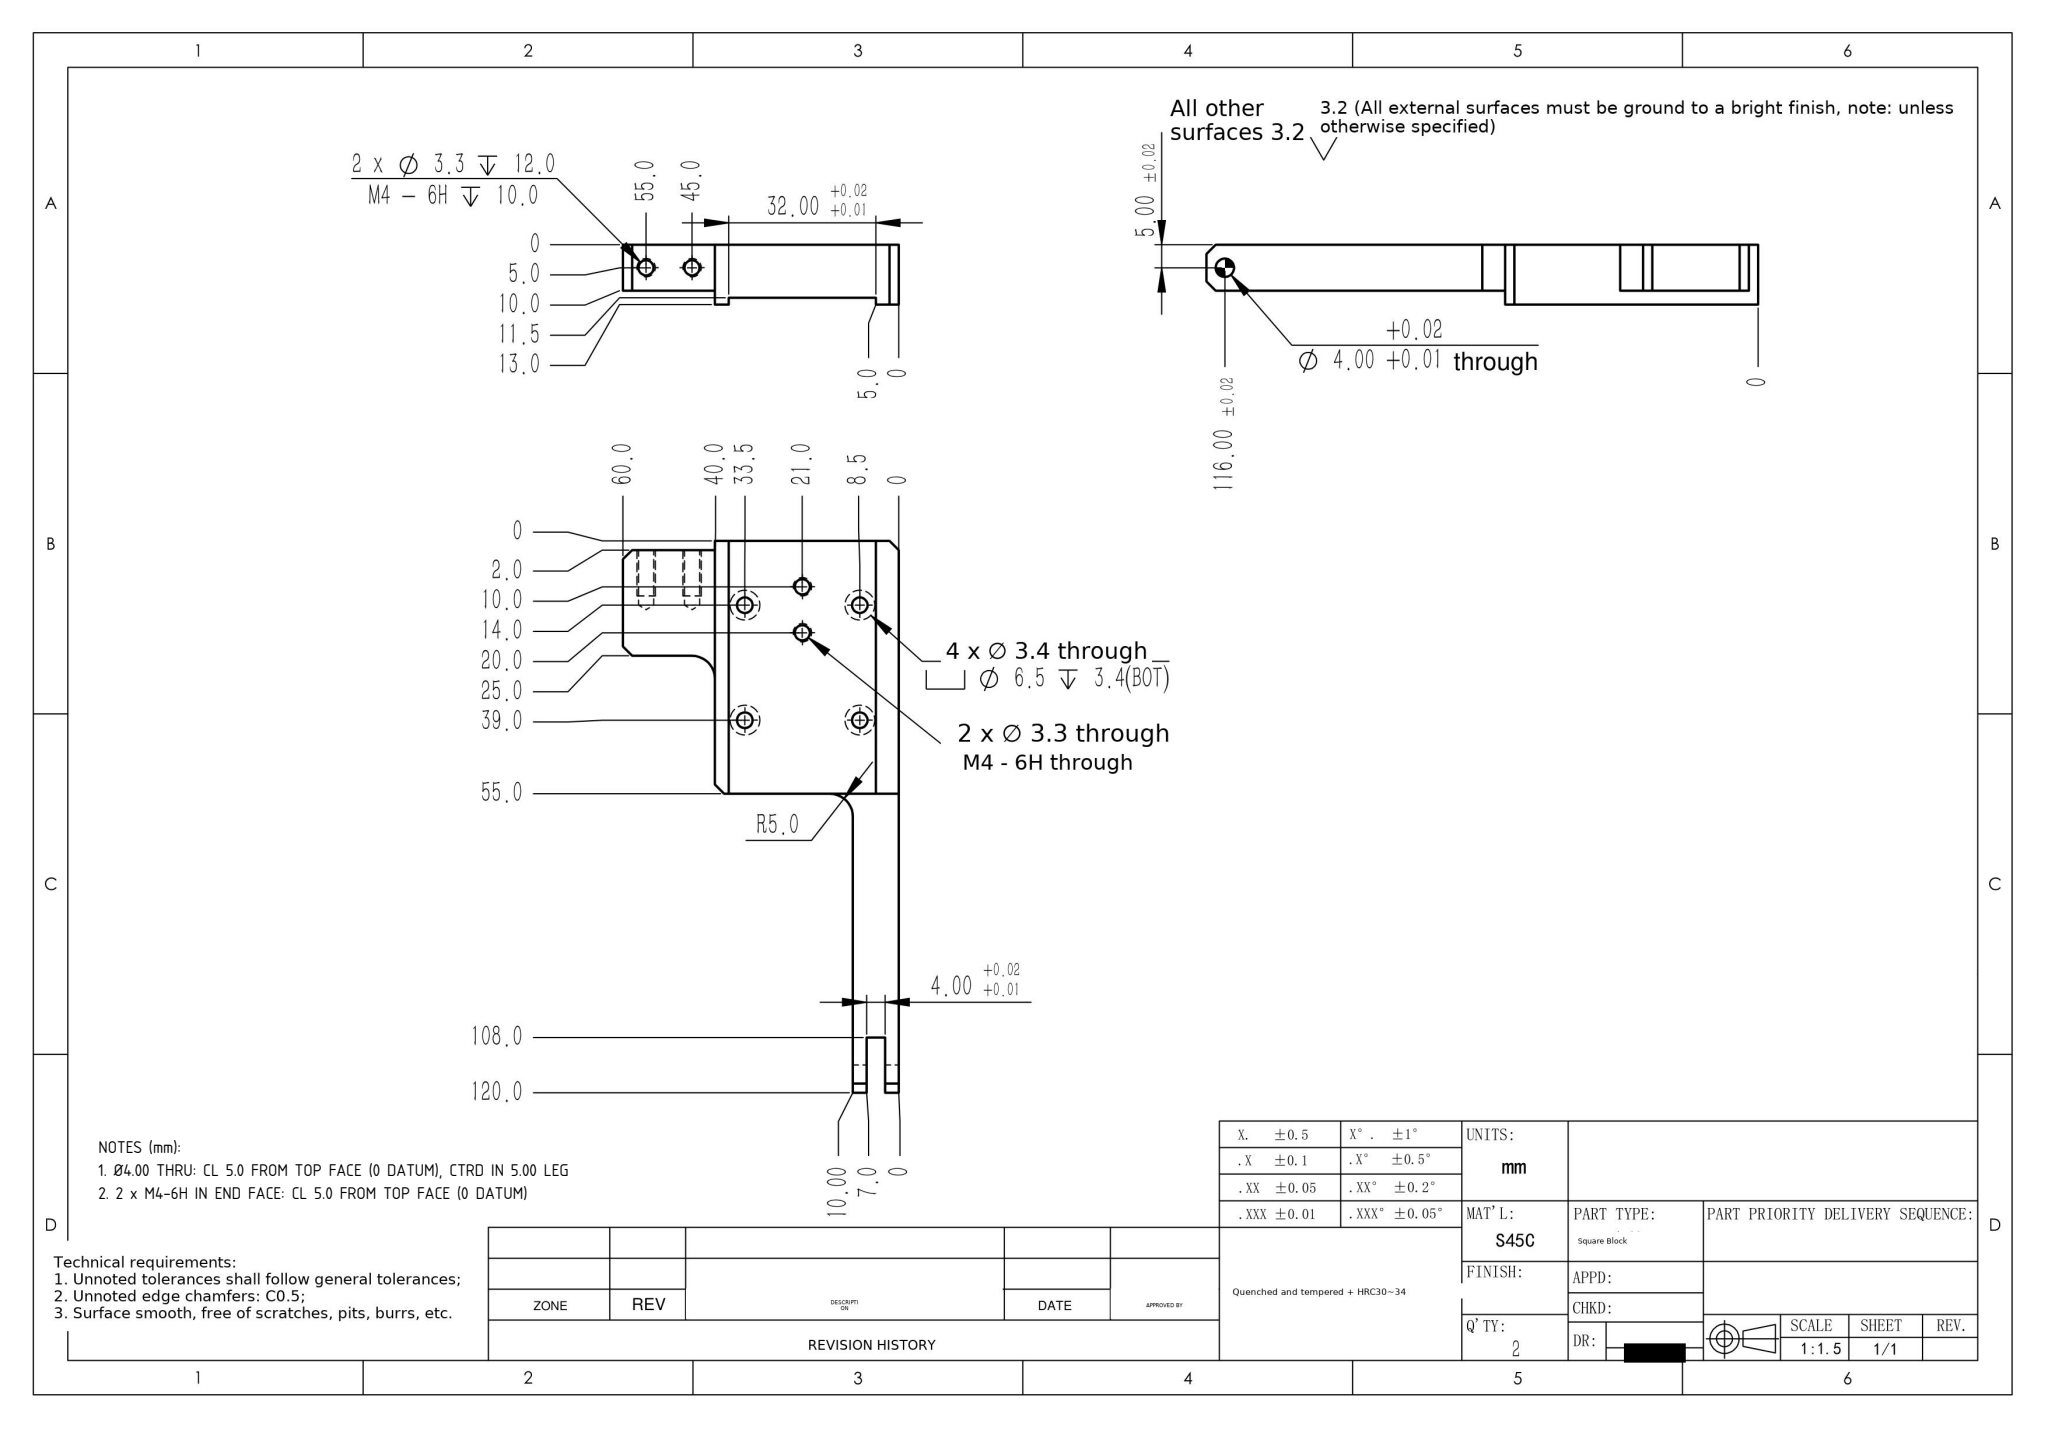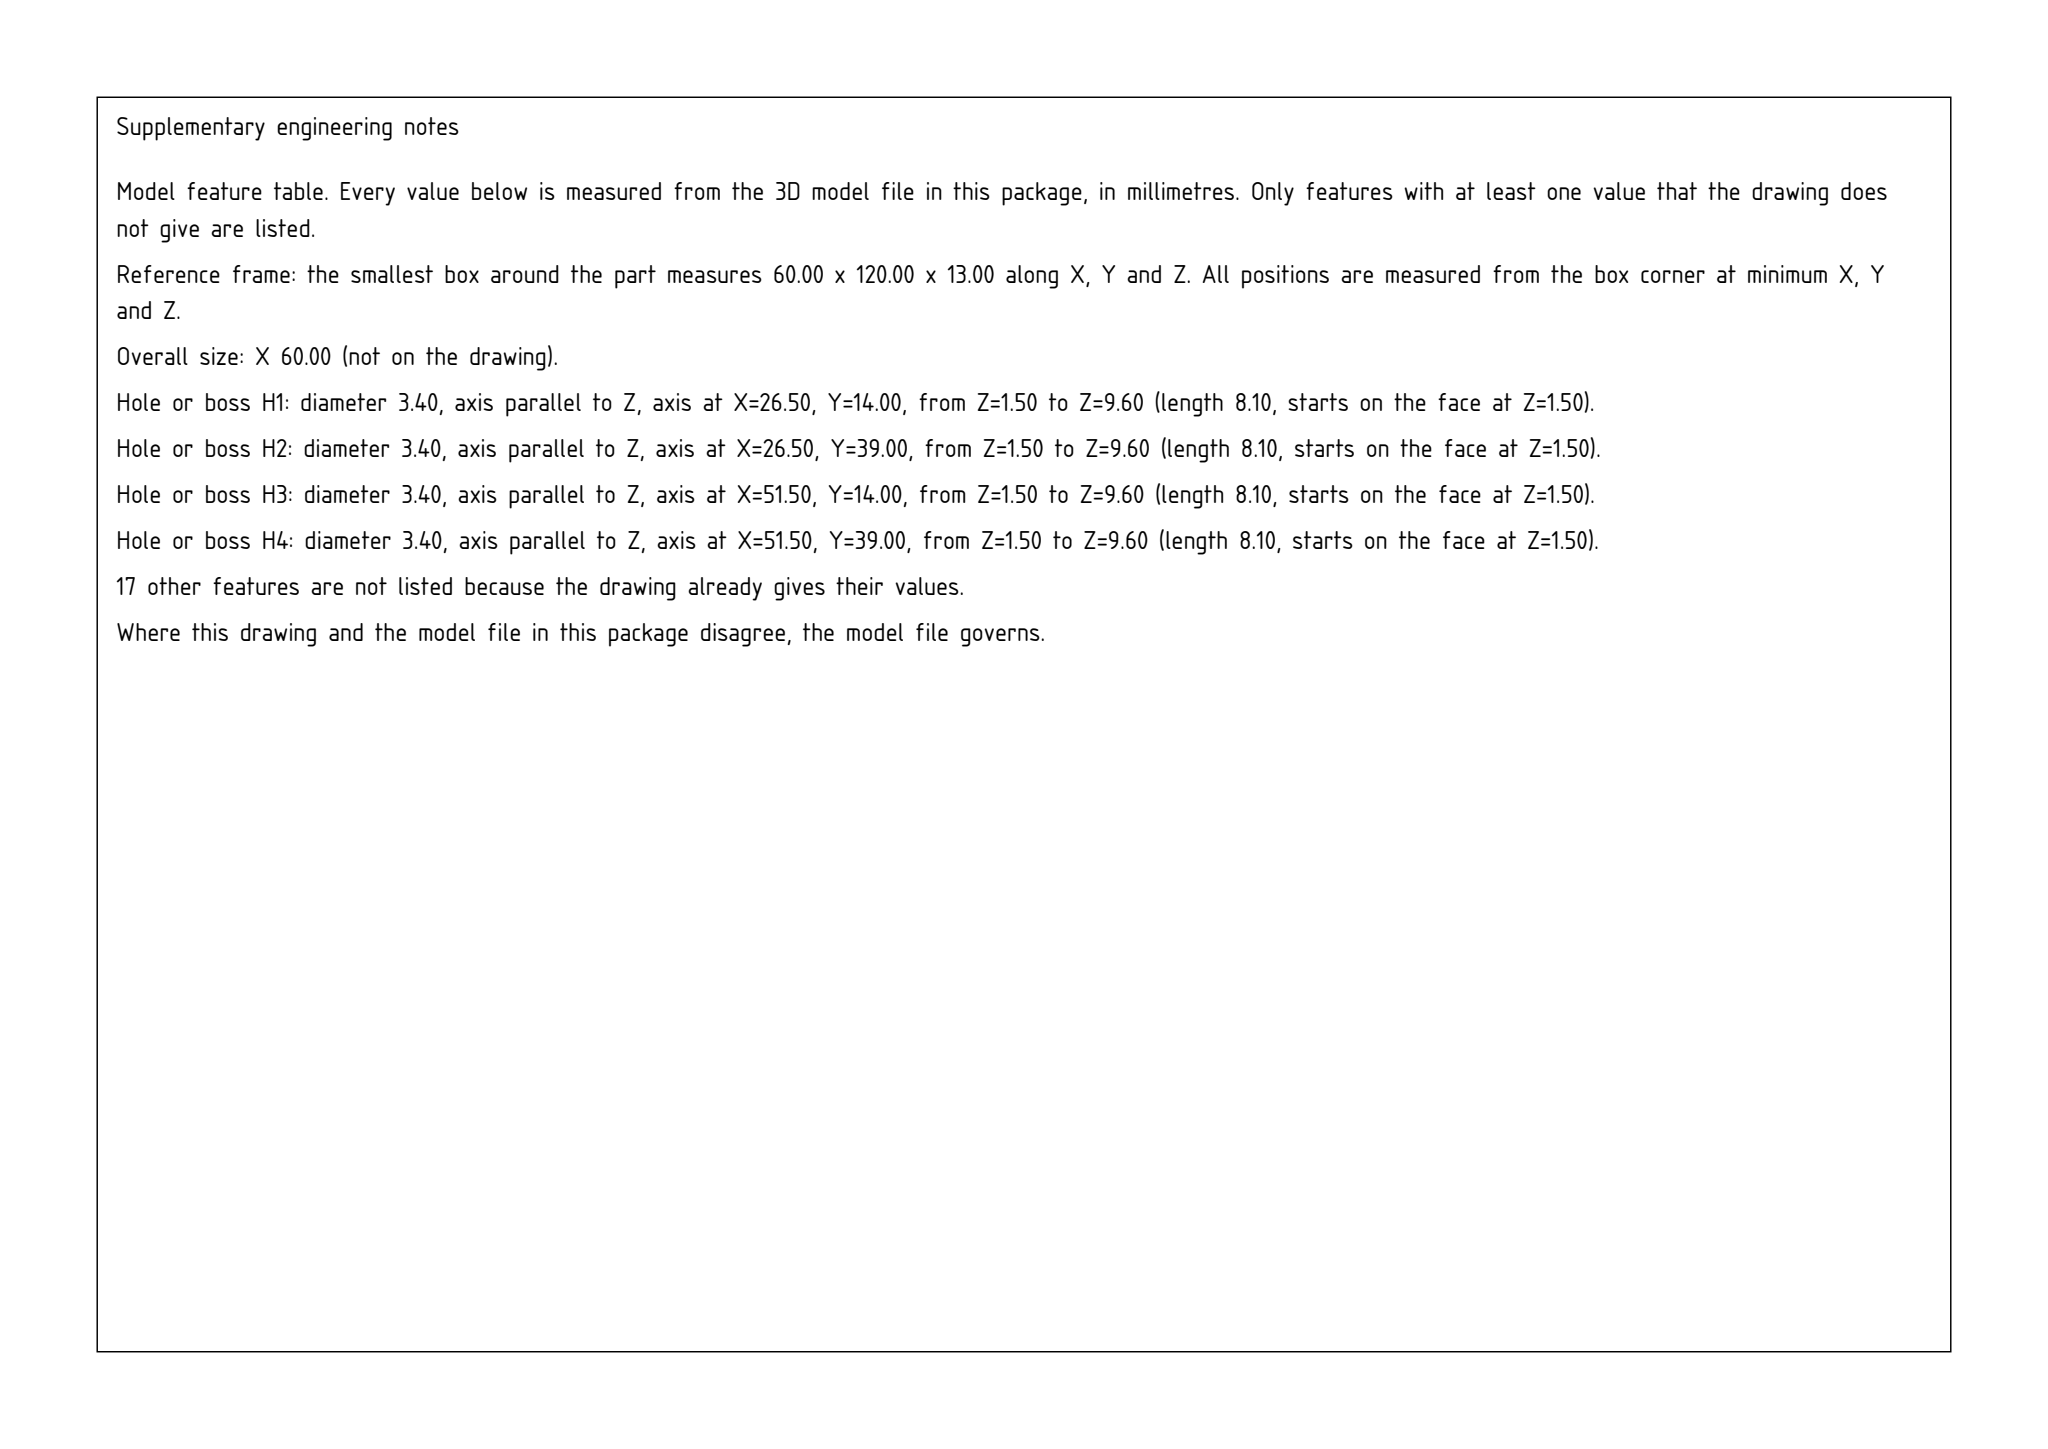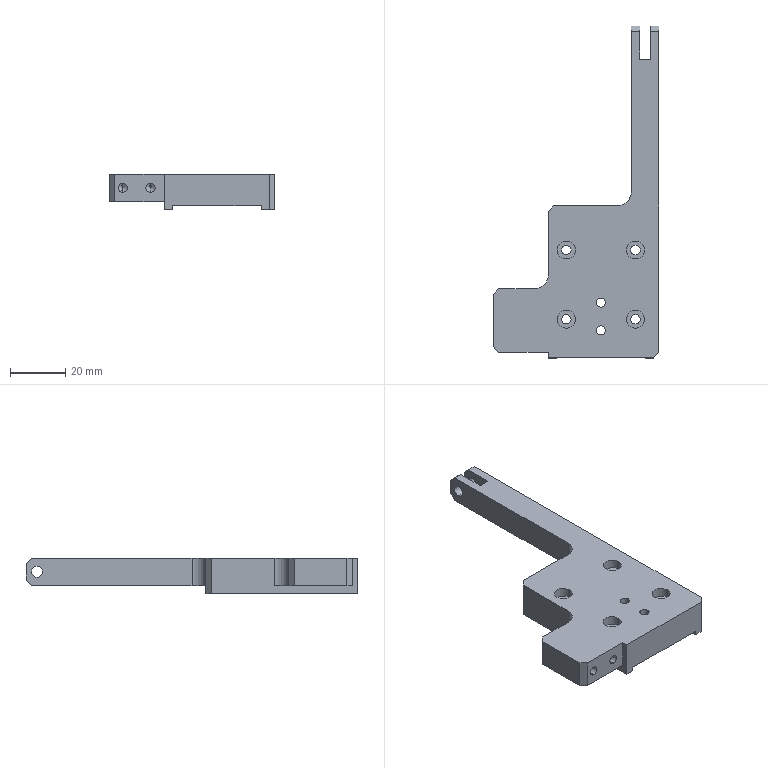Part | SolidWorks | mm | 1 solid | 67 faces | box 60 x 120 x 13 mm | volume 35343 mm3 | plane 33 | cylinder 30 | cone 4 | commonest cylinder face diameters 3.3 x8 6.5 x8 3.4 x8 4 x4 10 x2
Drawing notes:
Ø4.00 THRU: CL 5.0 FROM TOP FACE (0 DATUM), CTRD IN 5.00 LEG | from the solid: Ø4.0 cyl, axis x, y=116.0, z=8.0; top face z=13.0 -> 13.0-8.0=5.0; leg thk 5.00 (z 5.5-10.5) so on leg CL
2 x M4-6H IN END FACE: CL 5.0 FROM TOP FACE (0 DATUM) | from the solid: Ø3.3 cyls, axis y, z=8.0, top face z=13.0 -> 5.0; x=5.0 & 15.0 match 55.0/45.0 locs
build123d program:
from build123d import *

# Parameters (mm, degrees)
SKETCH1_W                                       = 60
SKETCH1_H                                       = 120
BOSS_EXTRUDE1_DEPTH                             = 13
SKETCH2_W                                       = 32
SKETCH2_H                                       = 80
CUT_EXTRUDE1_DEPTH                              = 1.5
M3_HEX_SOCKET_HEAD_CAP_SCREW_CBORE1_D           = 3.4
M3_HEX_SOCKET_HEAD_CAP_SCREW_CBORE1_CBORE_D     = 6.5
M3_HEX_SOCKET_HEAD_CAP_SCREW_CBORE1_CBORE_DEPTH = 3.4
CUT_EXTRUDE4_DEPTH                              = 125.374
SKETCH10_W                                      = 4
SKETCH10_H                                      = 12
CUT_EXTRUDE5_DEPTH                              = 125.374
SKETCH13_W                                      = 60
SKETCH13_H                                      = 65
SKETCH13_W_2                                    = 20
SKETCH13_H_2                                    = 25
CUT_EXTRUDE6_DEPTH                              = 3
SIZE_MM_DOWEL_HOLE1_D                           = 4
SKETCH14_W                                      = 20
SKETCH14_H                                      = 13
CUT_EXTRUDE7_DEPTH                              = 2
M4_TAPPED_HOLE1_D                               = 3.3
M4_TAPPED_HOLE1_DEPTH                           = 12
M4_TAPPED_HOLE1_TIP                             = 0.9914
M4_TAPPED_HOLE2_D                               = 3.3
FILLET1_R                                       = 5
CHAMFER2_SIZE                                   = 2


with BuildPart() as part:
    # Sketch1 → Boss-Extrude1 (new body)
    with BuildSketch(Plane.XY):
        with Locations((0, 60)):
            Rectangle(SKETCH1_W, SKETCH1_H)
    extrude(amount=BOSS_EXTRUDE1_DEPTH)

    # Sketch2 → Cut-Extrude1 (cut)
    with BuildSketch(Plane(origin=(0, 0, 0), x_dir=(-1, 0, 0), z_dir=(0, 0, -1))):
        with Locations((-9, 40)):
            Rectangle(SKETCH2_W, SKETCH2_H)
    extrude(amount=-CUT_EXTRUDE1_DEPTH, mode=Mode.SUBTRACT)

    # M3 Hex Socket Head Cap Screw CBORE1 (through all)
    with Locations(Plane.XY.offset(13)):
        with Locations((21.5, 14), (-3.5, 14), (-3.5, 39), (21.5, 39)):
            CounterBoreHole(M3_HEX_SOCKET_HEAD_CAP_SCREW_CBORE1_D / 2, M3_HEX_SOCKET_HEAD_CAP_SCREW_CBORE1_CBORE_D / 2, M3_HEX_SOCKET_HEAD_CAP_SCREW_CBORE1_CBORE_DEPTH)

    # Sketch9 → Cut-Extrude4 (cut, through all)
    with BuildSketch(Plane.XY.offset(13)):
        Polygon((-10, 55), (-10, 25), (-30, 25), (-30, 120), (20, 120), (20, 55), align=None)
    extrude(amount=-CUT_EXTRUDE4_DEPTH, mode=Mode.SUBTRACT)

    # Sketch10 → Cut-Extrude5 (cut, through all)
    with BuildSketch(Plane.XY.offset(13)):
        with Locations((25, 114)):
            Rectangle(SKETCH10_W, SKETCH10_H)
    extrude(amount=-CUT_EXTRUDE5_DEPTH, mode=Mode.SUBTRACT)

    # Sketch13 → Cut-Extrude6 (cut)
    with BuildSketch(Plane(origin=(0, 0, 0), x_dir=(-1, 0, 0), z_dir=(0, 0, -1))):
        with Locations((0, 87.5)):
            Rectangle(SKETCH13_W, SKETCH13_H)
        with Locations((20, 12.5)):
            Rectangle(SKETCH13_W_2, SKETCH13_H_2)
    extrude(amount=-CUT_EXTRUDE6_DEPTH, mode=Mode.SUBTRACT)

    # Size mm Dowel Hole1 (through all)
    with Locations(Plane(origin=(30, 0, 0), x_dir=(0, 0, -1), z_dir=(1, 0, 0))):
        with Locations((-8, 116)):
            Hole(SIZE_MM_DOWEL_HOLE1_D / 2)

    # Sketch14 → Cut-Extrude7 (cut)
    with BuildSketch(Plane.XZ):
        with Locations((-20, 6.5)):
            Rectangle(SKETCH14_W, SKETCH14_H)
    extrude(amount=-CUT_EXTRUDE7_DEPTH, mode=Mode.SUBTRACT)

    # M4 Tapped Hole1
    with Locations(Plane(origin=(0, 2, 0), x_dir=(-1, 0, 0), z_dir=(0, -1, 0))):
        with Locations((25, -8), (15, -8)):
            Hole(M4_TAPPED_HOLE1_D / 2, depth=M4_TAPPED_HOLE1_DEPTH)
            with Locations((0, 0, -(M4_TAPPED_HOLE1_DEPTH + M4_TAPPED_HOLE1_TIP / 2))):  # 118° drill point
                Cone(0, M4_TAPPED_HOLE1_D / 2, M4_TAPPED_HOLE1_TIP, mode=Mode.SUBTRACT)

    # M4 Tapped Hole2 (through all)
    with Locations(Plane.XY.offset(13)):
        with Locations((9, 20), (9, 10)):
            Hole(M4_TAPPED_HOLE2_D / 2)

    # Fillet1
    fillet1_edges = [part.edges().sort_by_distance(p)[0] for p in [
        (20, 55, 8),
        (-10, 25, 8),
    ]]
    fillet(fillet1_edges, radius=FILLET1_R)

    # Chamfer2
    chamfer2_edges = [part.edges().sort_by_distance(p)[0] for p in [
        (21.5, 120, 3),
        (28.5, 120, 3),
        (28.5, 120, 13),
        (-30, 25, 8),
        (-30, 2, 8),
        (-10, 55, 6.5),
        (30, 0, 6.5),
        (21.5, 120, 13),
    ]]
    chamfer(chamfer2_edges, length=CHAMFER2_SIZE)


solid = part.part